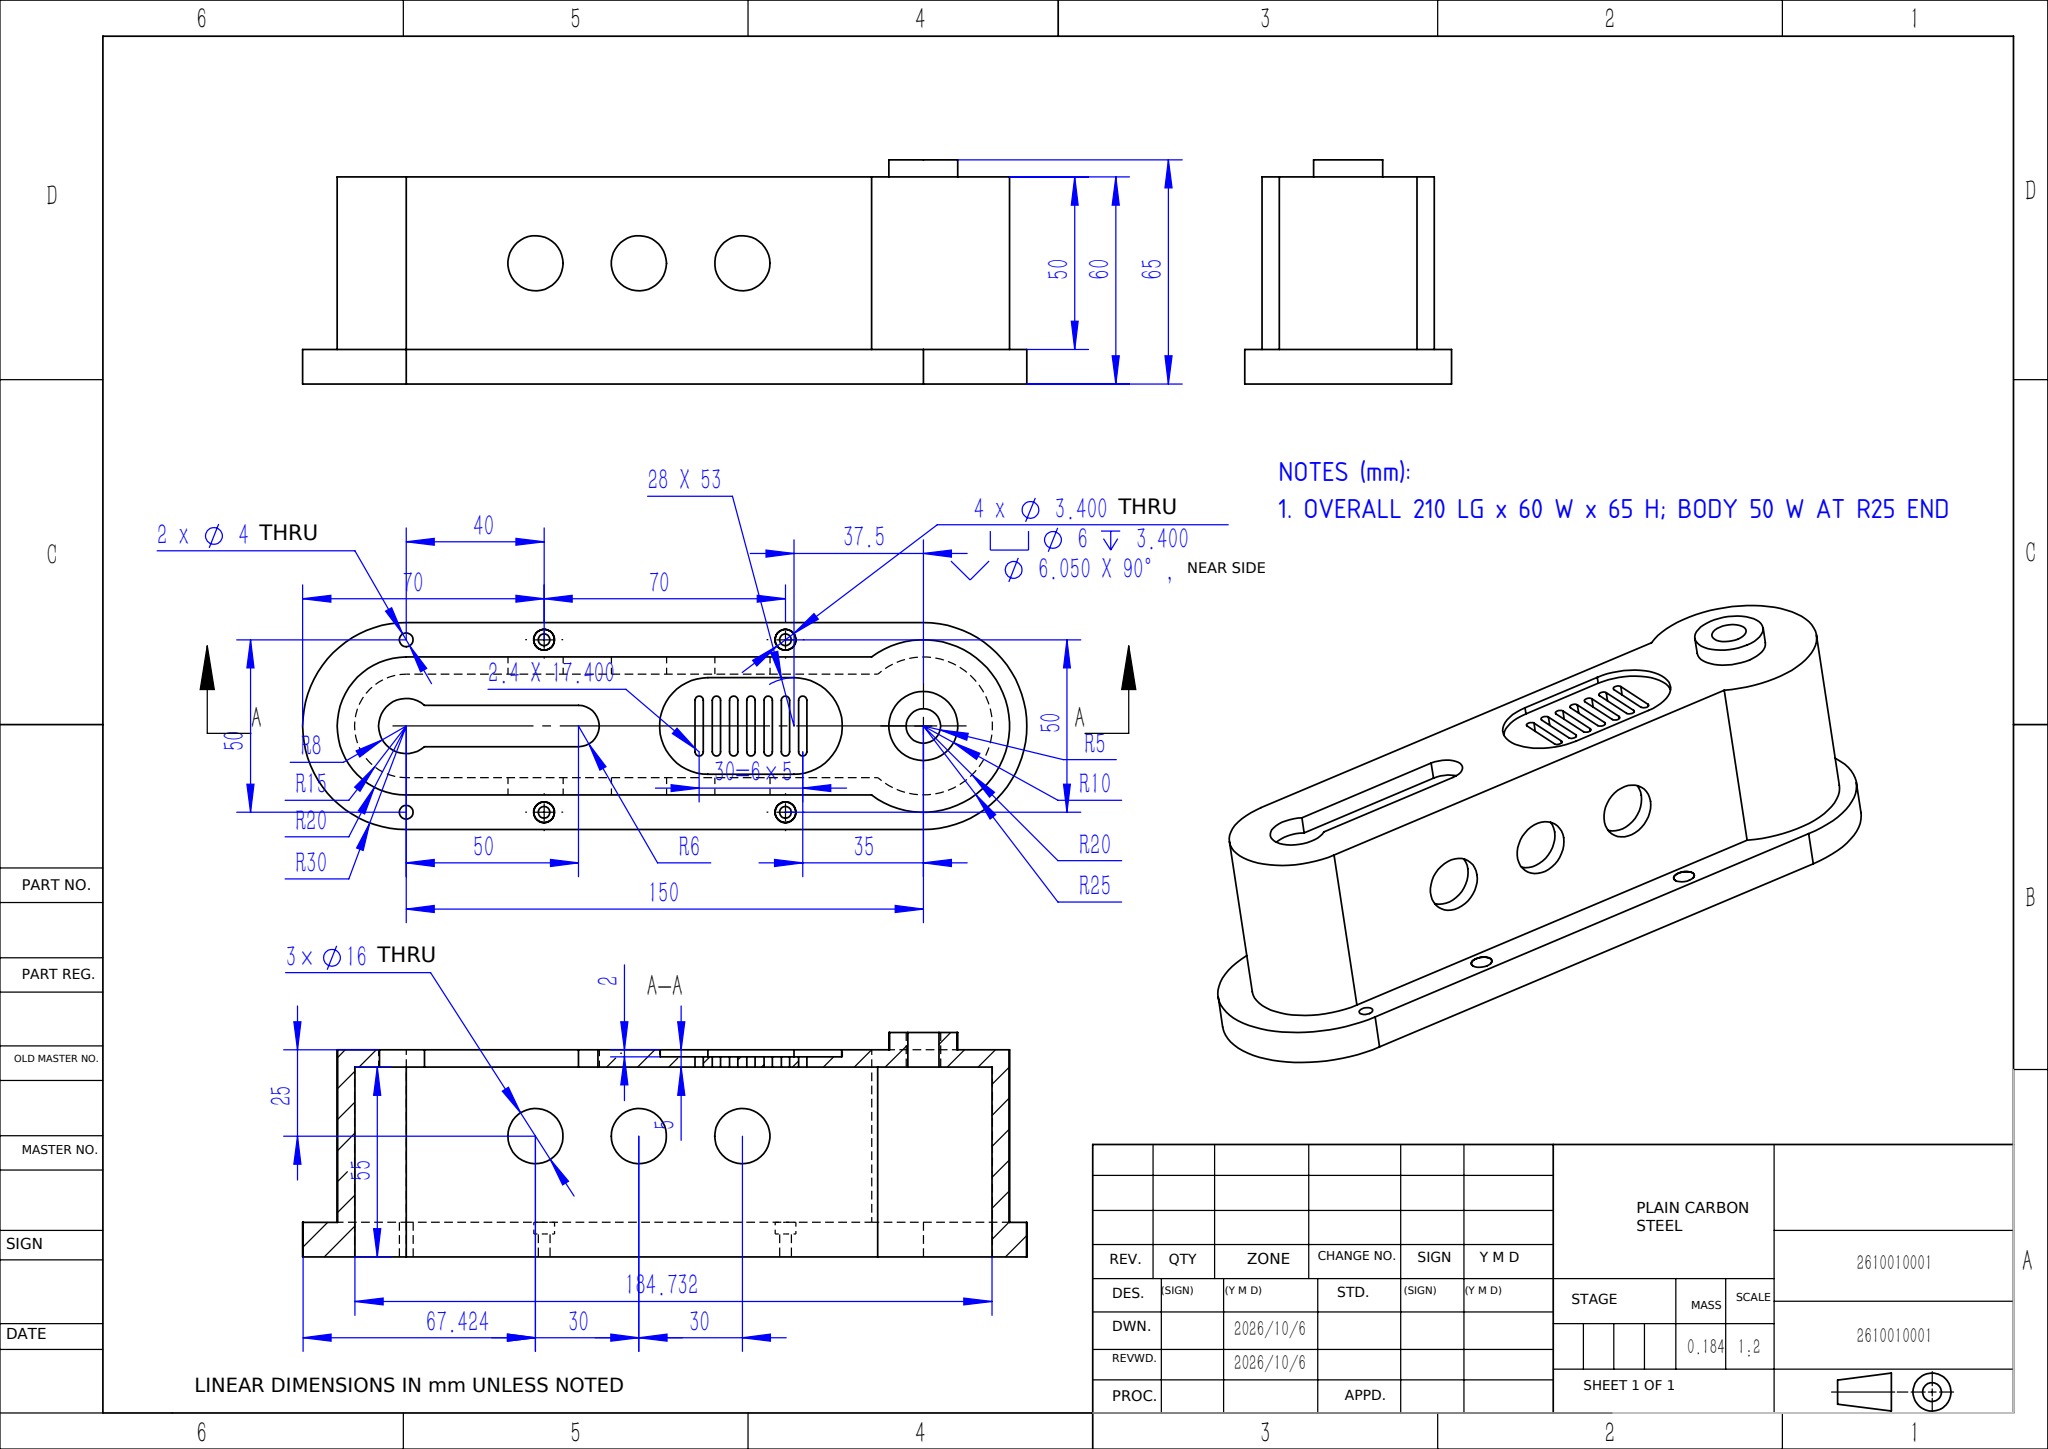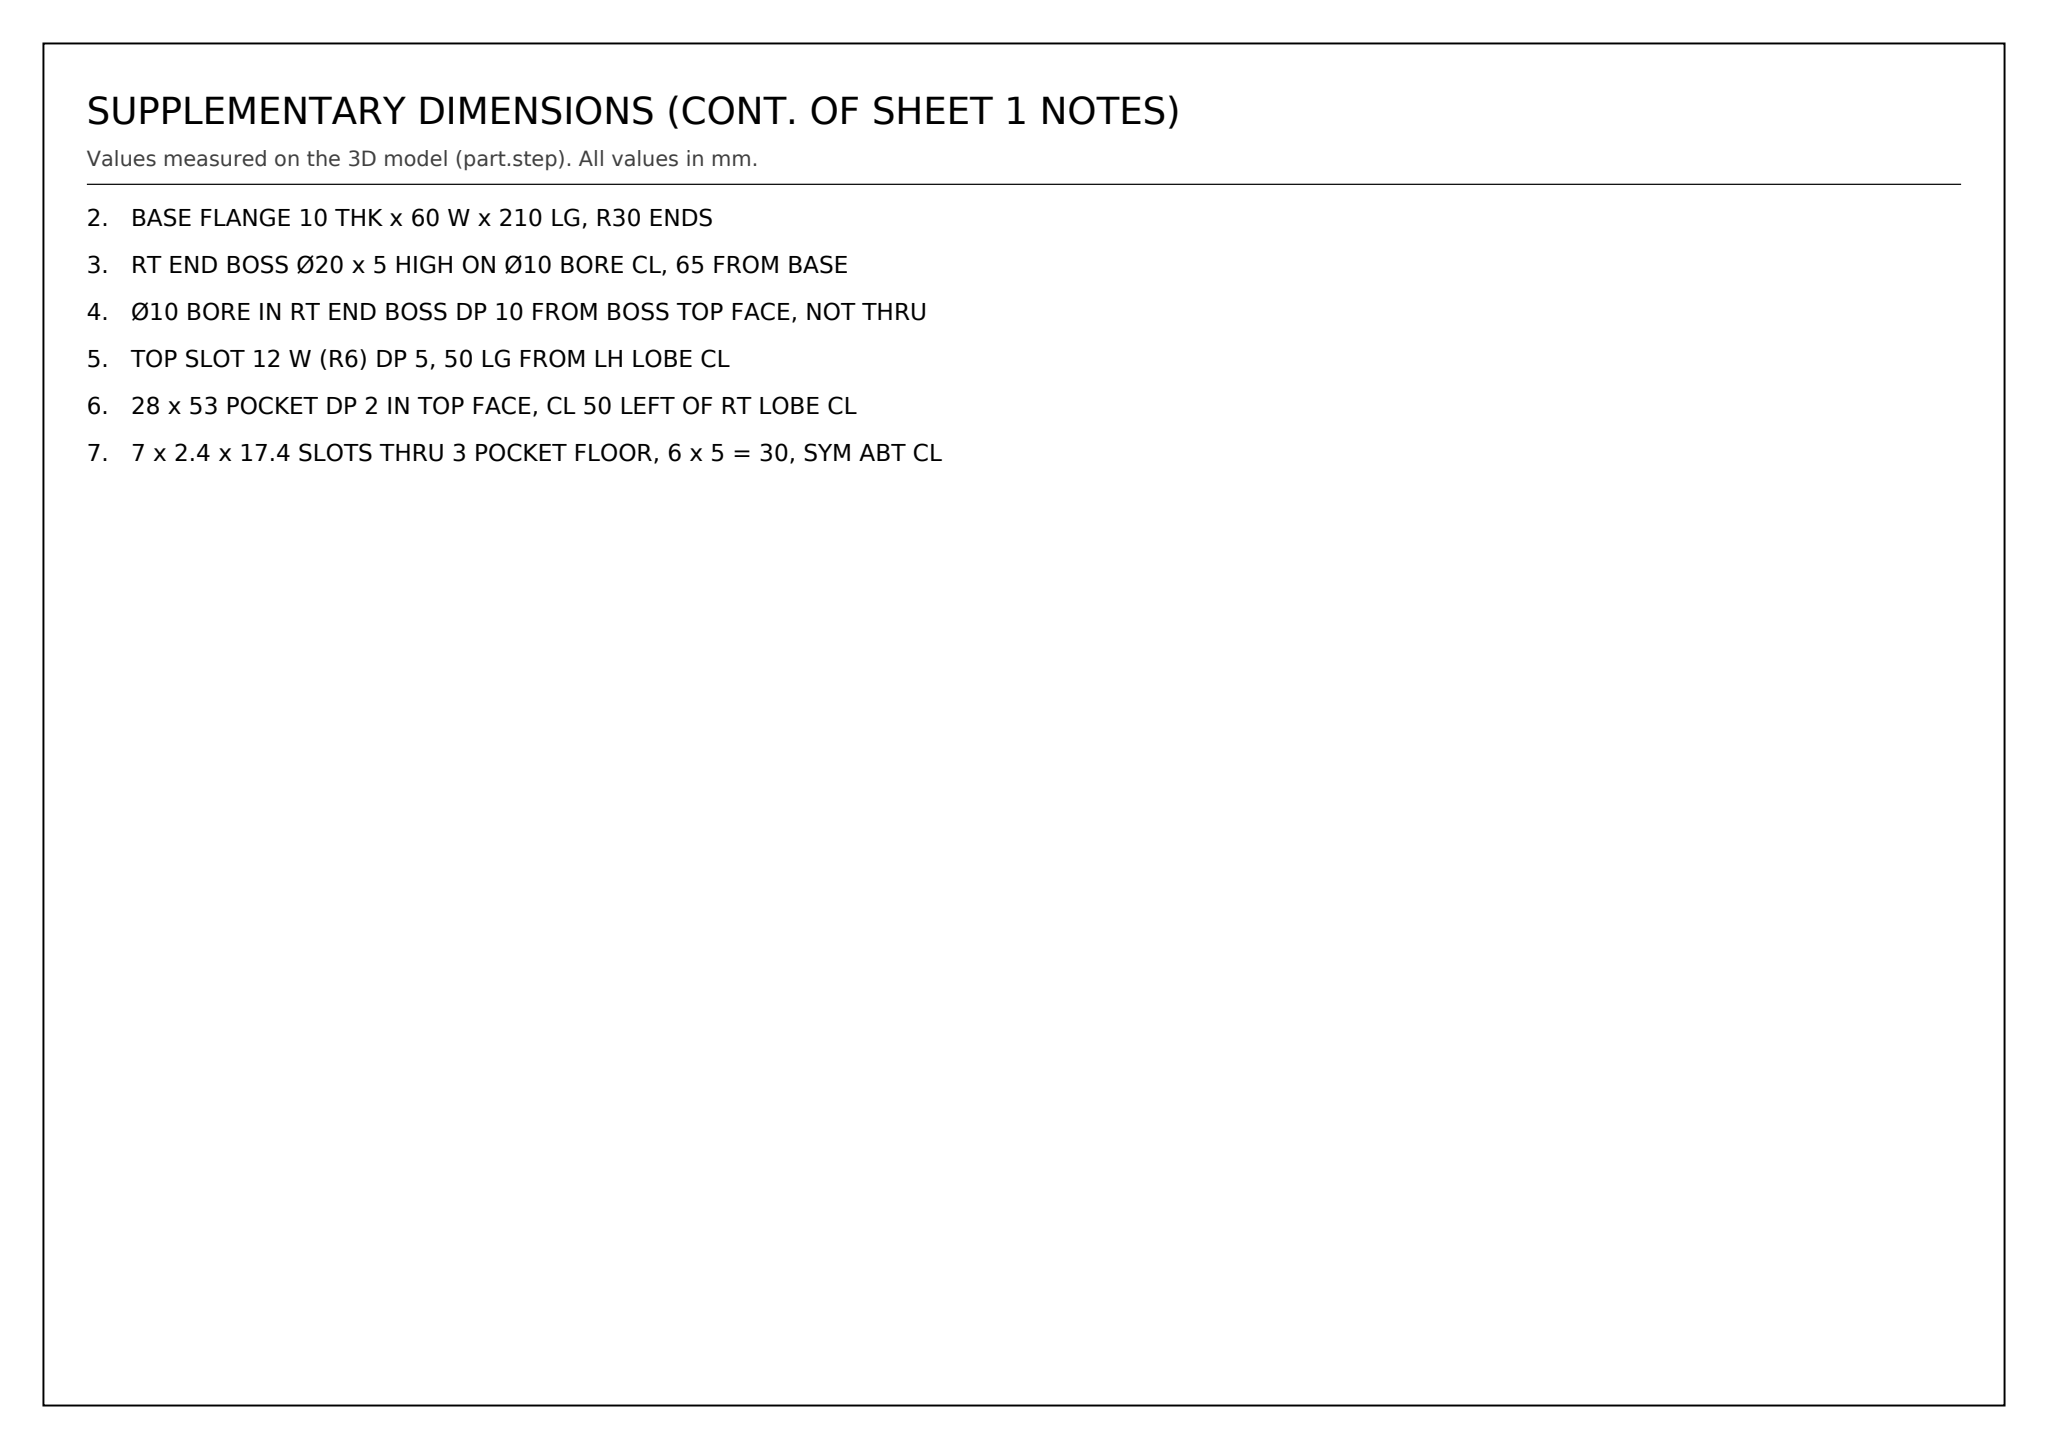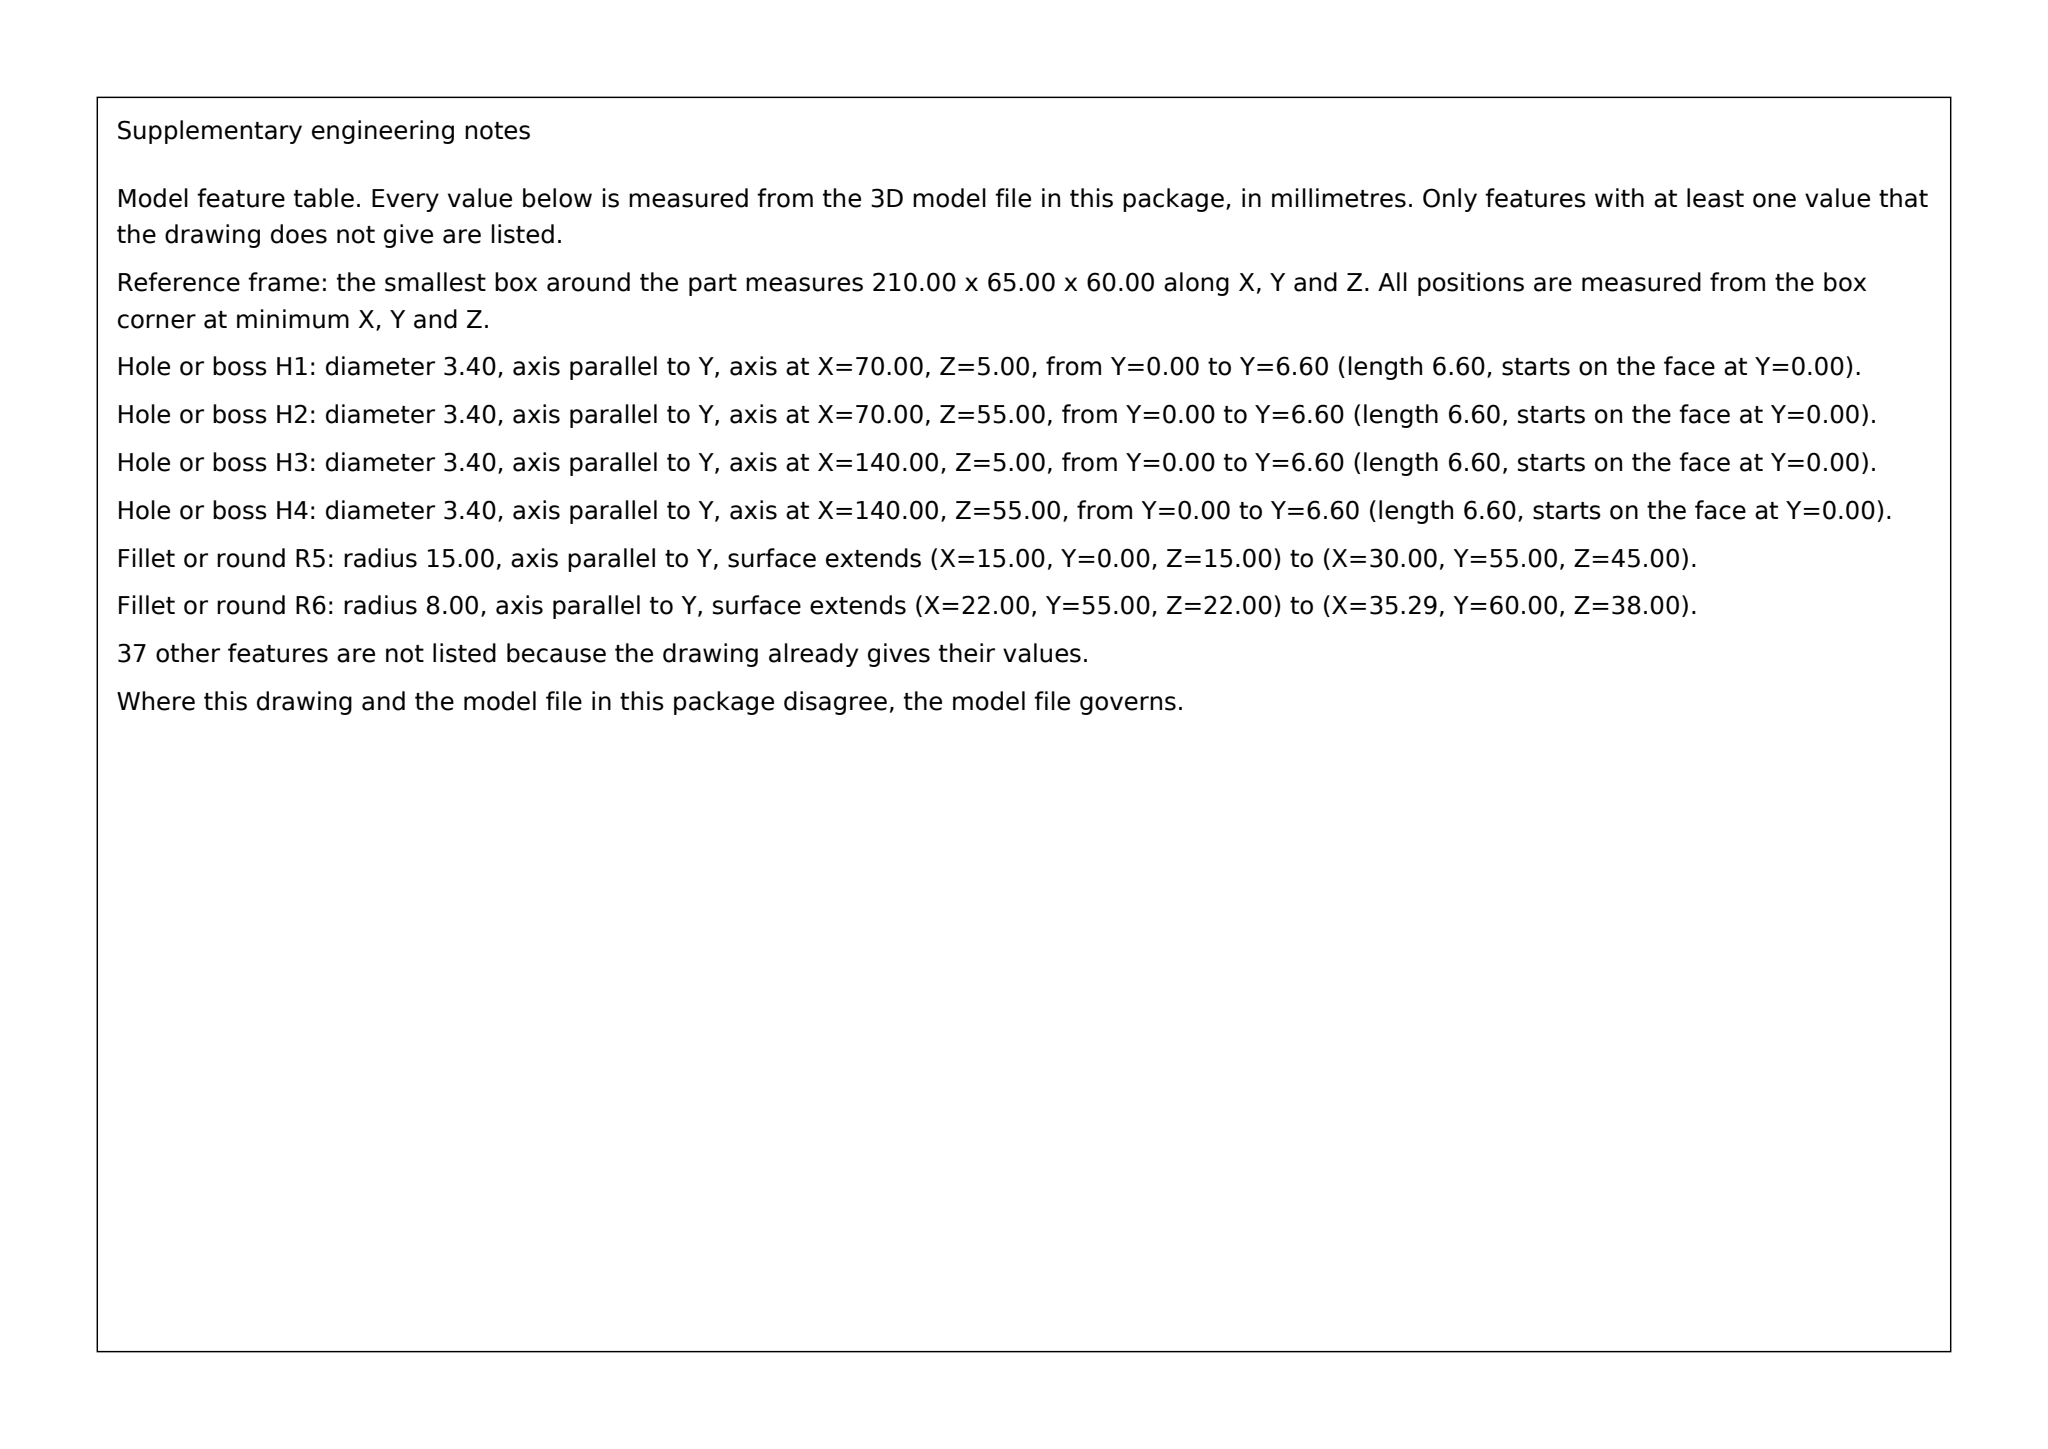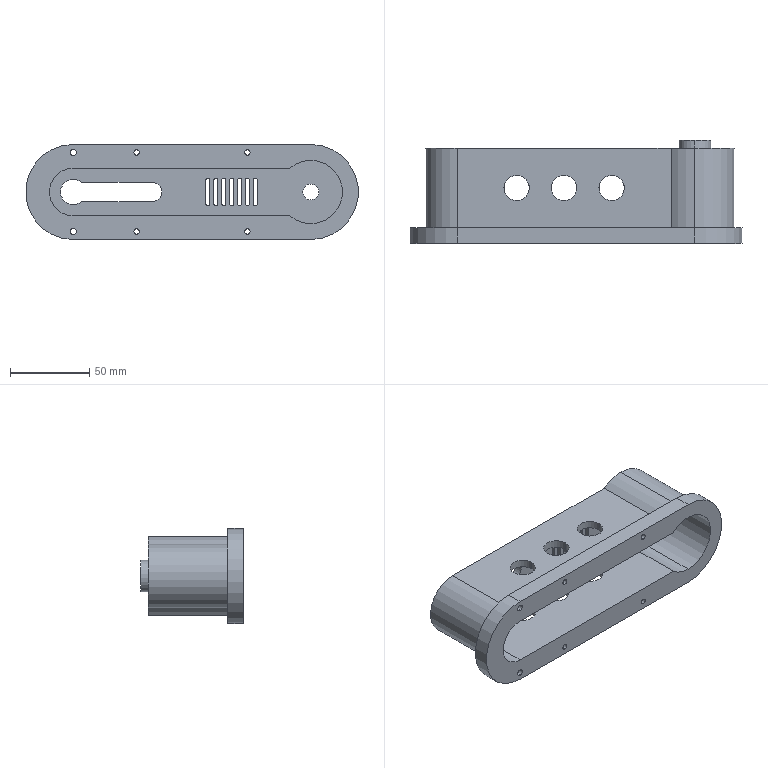Part | SolidWorks | mm | 1 solid | 115 faces | box 210 x 65 x 60 mm | volume 183942 mm3 | cylinder 73 | plane 34 | cone 8 | commonest cylinder face diameters 2.4 x21 16 x15 6 x8 3.4 x8 4 x4 40 x4 50 x3 10 x2
Drawing notes:
OVERALL 210 LG x 60 W x 65 H; BODY 50 W AT R25 END | from the solid: bbox 210 x 65 x 60; Ø60 and Ø50 y-cyls at z=30
BASE FLANGE 10 THK x 60 W x 210 LG, R30 ENDS | from the solid: Ø60 y-cyl len 10 at x=30 & x=180; y planes 0/10; bbox X=210
RT END BOSS Ø20 x 5 HIGH ON Ø10 BORE CL, 65 FROM BASE | from the solid: Ø20 y-cyl len 5 at x=180,z=30; y planes 60/65
Ø10 BORE IN RT END BOSS DP 10 FROM BOSS TOP FACE, NOT THRU | from the solid: cyl [10,"y",[180,null,30],len 10]; bore y=55..65
TOP SLOT 12 W (R6) DP 5, 50 LG FROM LH LOBE CL | from the solid: Ø12 y-cyl len 5 at x=80 and Ø16 y-cyl len 5 at x=30, z=30; y 55-60
28 x 53 POCKET DP 2 IN TOP FACE, CL 50 LEFT OF RT LOBE CL | from the solid: Ø28 y-cyls len 2 at x=117.5 & 142.5, z=30; y 58-60; CL x=130 vs 180
7 x 2.4 x 17.4 SLOTS THRU 3 POCKET FLOOR, 6 x 5 = 30, SYM ABT CL | from the solid: Ø2.4 y-cyls len 3 at x=115..145 step 5, z=22.5/37.5; y 55-58
build123d program:
from build123d import *

# Parameters (mm, degrees)
BOSS_EXTRUDE1_DEPTH                            = 10
BOSS_EXTRUDE2_DEPTH                            = 50
SKETCH4_R                                      = 10
BOSS_EXTRUDE3_DEPTH                            = 5
SKETCH5_R                                      = 5
CUT_EXTRUDE1_DEPTH                             = 128.083
CUT_EXTRUDE2_START                             = -5
CUT_EXTRUDE2_DEPTH                             = 120.599
M3_HEX_SOCKET_HEAD_CAP_SCREW_CBORE1_AT_2_COUNT = 2
M3_HEX_SOCKET_HEAD_CAP_SCREW_CBORE1_AT_2_PITCH = 70
M3_HEX_SOCKET_HEAD_CAP_SCREW_CBORE1_AT_3_COUNT = 2
M3_HEX_SOCKET_HEAD_CAP_SCREW_CBORE1_AT_3_PITCH = 50
M3_HEX_SOCKET_HEAD_CAP_SCREW_CBORE1_AT_4_COUNT = 2
M3_HEX_SOCKET_HEAD_CAP_SCREW_CBORE1_AT_4_PITCH = 86.023
CUT_EXTRUDE3_DEPTH                             = 125.599
CUT_EXTRUDE4_DEPTH                             = 2
CUT_EXTRUDE6_REACH                             = 125.649
F_4_0_4_DIAMETER_HOLE1_D                       = 4
SKETCH18_R                                     = 8
CUT_EXTRUDE7_DEPTH                             = 134.229


with BuildPart() as part:
    # Sketch1 → Boss-Extrude1 (new body)
    with BuildSketch(Plane(origin=(0, 0, 0), x_dir=(1, 0, 0), z_dir=(0, 1, 0))):
        with BuildLine():
            Line((-75, 30), (75, 30))
            ThreePointArc((75, 30), (105, 0), (75, -30))
            Line((75, -30), (-75, -30))
            ThreePointArc((-75, -30), (-105, 0), (-75, 30))
        make_face()
    extrude(amount=BOSS_EXTRUDE1_DEPTH)

    # Sketch2 → Boss-Extrude2 (add)
    with BuildSketch(Plane(origin=(0, 10, 0), x_dir=(1, 0, 0), z_dir=(0, 1, 0))):
        with BuildLine():
            Line((-75, -20), (60, -20))
            ThreePointArc((60, -20), (100, 0), (60, 20))
            Line((60, 20), (-75, 20))
            ThreePointArc((-75, 20), (-95, 0), (-75, -20))
        make_face()
    extrude(amount=BOSS_EXTRUDE2_DEPTH)

    # Sketch4 → Boss-Extrude3 (add)
    with BuildSketch(Plane(origin=(0, 60, 0), x_dir=(1, 0, 0), z_dir=(0, 1, 0))):
        with Locations(Location((75, 0, 0), (0, 0, 270))):
            Circle(SKETCH4_R)
    extrude(amount=BOSS_EXTRUDE3_DEPTH)

    # Sketch5 → Cut-Extrude1 (cut, through all)
    with BuildSketch(Plane(origin=(0, 65, 0), x_dir=(1, 0, 0), z_dir=(0, 1, 0))):
        with Locations(Location((75, 0, 0), (0, 0, 270))):
            Circle(SKETCH5_R)
    extrude(amount=-CUT_EXTRUDE1_DEPTH, mode=Mode.SUBTRACT)

    # Sketch6 → Cut-Extrude2 (cut, through all)
    with BuildSketch(Plane(origin=(0, 60, 0), x_dir=(1, 0, 0), z_dir=(0, 1, 0)).offset(CUT_EXTRUDE2_START)):
        with BuildLine():
            Line((61.771, 15), (-75, 15))
            ThreePointArc((-75, 15), (-90, 0), (-75, -15))
            Line((-75, -15), (61.771, -15))
            ThreePointArc((61.771, -15), (95, 0), (61.771, 15))
        make_face()
    extrude(amount=-CUT_EXTRUDE2_DEPTH, mode=Mode.SUBTRACT)

    # Sketch8 → M3 Hex Socket Head Cap Screw CBORE1 (revolve, cut)
    with BuildSketch(Plane(origin=(-35, 10, 25), x_dir=(0, 0, 1), z_dir=(1, 0, 0))):
        Polygon((0, 0), (0, 10), (1.7, 10), (1.7, 3.4), (3, 3.4), (3, 0.025), (3.025, 0), align=None)
    m3_hex_socket_head_cap_screw_cbore1 = revolve(axis=Axis((-35, 16.35, 25), (0, -1, 0)), mode=Mode.SUBTRACT)

    # M3 Hex Socket Head Cap Screw CBORE1 at 2: M3 Hex Socket Head Cap Screw CBORE1 ×2
    with Locations(*[(i * M3_HEX_SOCKET_HEAD_CAP_SCREW_CBORE1_AT_2_PITCH, 0, 0) for i in range(1, M3_HEX_SOCKET_HEAD_CAP_SCREW_CBORE1_AT_2_COUNT)]):
        add(m3_hex_socket_head_cap_screw_cbore1, mode=Mode.SUBTRACT)

    # M3 Hex Socket Head Cap Screw CBORE1 at 3: M3 Hex Socket Head Cap Screw CBORE1 ×2
    with Locations(*[(0, 0, -i * M3_HEX_SOCKET_HEAD_CAP_SCREW_CBORE1_AT_3_PITCH) for i in range(1, M3_HEX_SOCKET_HEAD_CAP_SCREW_CBORE1_AT_3_COUNT)]):
        add(m3_hex_socket_head_cap_screw_cbore1, mode=Mode.SUBTRACT)

    # M3 Hex Socket Head Cap Screw CBORE1 at 4: M3 Hex Socket Head Cap Screw CBORE1 ×2
    with Locations(*[Vector(0.8137, 0, -0.5812) * (i * M3_HEX_SOCKET_HEAD_CAP_SCREW_CBORE1_AT_4_PITCH) for i in range(1, M3_HEX_SOCKET_HEAD_CAP_SCREW_CBORE1_AT_4_COUNT)]):
        add(m3_hex_socket_head_cap_screw_cbore1, mode=Mode.SUBTRACT)

    # Sketch12 → Cut-Extrude3 (cut, through all)
    with BuildSketch(Plane(origin=(0, 60, 0), x_dir=(1, 0, 0), z_dir=(0, 1, 0))):
        with BuildLine():
            Line((-69.708, 6), (-25, 6))
            ThreePointArc((-25, 6), (-19, 0), (-25, -6))
            Line((-25, -6), (-69.708, -6))
            ThreePointArc((-69.708, -6), (-83, 0), (-69.708, 6))
        make_face()
    extrude(amount=-CUT_EXTRUDE3_DEPTH, mode=Mode.SUBTRACT)

    # Sketch13 → Cut-Extrude4 (cut)
    with BuildSketch(Plane(origin=(0, 60, 0), x_dir=(1, 0, 0), z_dir=(0, 1, 0))):
        with BuildLine():
            Line((12.5, 14), (37.5, 14))
            ThreePointArc((37.5, 14), (51.5, 0), (37.5, -14))
            Line((37.5, -14), (12.5, -14))
            ThreePointArc((12.5, -14), (-1.5, 0), (12.5, 14))
        make_face()
    extrude(amount=-CUT_EXTRUDE4_DEPTH, mode=Mode.SUBTRACT)

    # Sketch14 → Cut-Extrude6 (cut, up to next)
    with BuildSketch(Plane(origin=(0, 58, 0), x_dir=(1, 0, 0), z_dir=(0, 1, 0)), mode=Mode.PRIVATE) as cut_extrude6_sk1:
        with BuildLine():
            Line((41.2, 7.5), (41.2, -7.5))
            ThreePointArc((41.2, -7.5), (40, -8.7), (38.8, -7.5))
            Line((38.8, -7.5), (38.8, 7.5))
            ThreePointArc((38.8, 7.5), (40, 8.7), (41.2, 7.5))
        make_face()
    cut_extrude6_tool1 = extrude(cut_extrude6_sk1.sketch, amount=-CUT_EXTRUDE6_REACH, mode=Mode.PRIVATE) & part.part
    # Sketch14 → Cut-Extrude6 (cut, up to next)
    with BuildSketch(Plane(origin=(0, 58, 0), x_dir=(1, 0, 0), z_dir=(0, 1, 0)), mode=Mode.PRIVATE) as cut_extrude6_sk2:
        with BuildLine():
            Line((36.2, 7.5), (36.2, -7.5))
            ThreePointArc((36.2, -7.5), (35, -8.7), (33.8, -7.5))
            Line((33.8, -7.5), (33.8, 7.5))
            ThreePointArc((33.8, 7.5), (35, 8.7), (36.2, 7.5))
        make_face()
    cut_extrude6_tool2 = extrude(cut_extrude6_sk2.sketch, amount=-CUT_EXTRUDE6_REACH, mode=Mode.PRIVATE) & part.part
    # Sketch14 → Cut-Extrude6 (cut, up to next)
    with BuildSketch(Plane(origin=(0, 58, 0), x_dir=(1, 0, 0), z_dir=(0, 1, 0)), mode=Mode.PRIVATE) as cut_extrude6_sk3:
        with BuildLine():
            Line((31.2, 7.5), (31.2, -7.5))
            ThreePointArc((31.2, -7.5), (30, -8.7), (28.8, -7.5))
            Line((28.8, -7.5), (28.8, 7.5))
            ThreePointArc((28.8, 7.5), (30, 8.7), (31.2, 7.5))
        make_face()
    cut_extrude6_tool3 = extrude(cut_extrude6_sk3.sketch, amount=-CUT_EXTRUDE6_REACH, mode=Mode.PRIVATE) & part.part
    # Sketch14 → Cut-Extrude6 (cut, up to next)
    with BuildSketch(Plane(origin=(0, 58, 0), x_dir=(1, 0, 0), z_dir=(0, 1, 0)), mode=Mode.PRIVATE) as cut_extrude6_sk4:
        with BuildLine():
            Line((26.2, 7.5), (26.2, -7.5))
            ThreePointArc((26.2, -7.5), (25, -8.7), (23.8, -7.5))
            Line((23.8, -7.5), (23.8, 7.5))
            ThreePointArc((23.8, 7.5), (25, 8.7), (26.2, 7.5))
        make_face()
    cut_extrude6_tool4 = extrude(cut_extrude6_sk4.sketch, amount=-CUT_EXTRUDE6_REACH, mode=Mode.PRIVATE) & part.part
    # Sketch14 → Cut-Extrude6 (cut, up to next)
    with BuildSketch(Plane(origin=(0, 58, 0), x_dir=(1, 0, 0), z_dir=(0, 1, 0)), mode=Mode.PRIVATE) as cut_extrude6_sk5:
        with BuildLine():
            Line((21.2, 7.5), (21.2, -7.5))
            ThreePointArc((21.2, -7.5), (20, -8.7), (18.8, -7.5))
            Line((18.8, -7.5), (18.8, 7.5))
            ThreePointArc((18.8, 7.5), (20, 8.7), (21.2, 7.5))
        make_face()
    cut_extrude6_tool5 = extrude(cut_extrude6_sk5.sketch, amount=-CUT_EXTRUDE6_REACH, mode=Mode.PRIVATE) & part.part
    # Sketch14 → Cut-Extrude6 (cut, up to next)
    with BuildSketch(Plane(origin=(0, 58, 0), x_dir=(1, 0, 0), z_dir=(0, 1, 0)), mode=Mode.PRIVATE) as cut_extrude6_sk6:
        with BuildLine():
            Line((16.2, 7.5), (16.2, -7.5))
            ThreePointArc((16.2, -7.5), (15, -8.7), (13.8, -7.5))
            Line((13.8, -7.5), (13.8, 7.5))
            ThreePointArc((13.8, 7.5), (15, 8.7), (16.2, 7.5))
        make_face()
    cut_extrude6_tool6 = extrude(cut_extrude6_sk6.sketch, amount=-CUT_EXTRUDE6_REACH, mode=Mode.PRIVATE) & part.part
    # Sketch14 → Cut-Extrude6 (cut, up to next)
    with BuildSketch(Plane(origin=(0, 58, 0), x_dir=(1, 0, 0), z_dir=(0, 1, 0)), mode=Mode.PRIVATE) as cut_extrude6_sk7:
        with BuildLine():
            Line((11.2, 7.5), (11.2, -7.5))
            ThreePointArc((11.2, -7.5), (10, -8.7), (8.8, -7.5))
            Line((8.8, -7.5), (8.8, 7.5))
            ThreePointArc((8.8, 7.5), (10, 8.7), (11.2, 7.5))
        make_face()
    cut_extrude6_tool7 = extrude(cut_extrude6_sk7.sketch, amount=-CUT_EXTRUDE6_REACH, mode=Mode.PRIVATE) & part.part
    add(cut_extrude6_tool1.solids().sort_by_distance((40, 58, 0))[0], mode=Mode.SUBTRACT)
    add(cut_extrude6_tool2.solids().sort_by_distance((35, 58, 0))[0], mode=Mode.SUBTRACT)
    add(cut_extrude6_tool3.solids().sort_by_distance((30, 58, 0))[0], mode=Mode.SUBTRACT)
    add(cut_extrude6_tool4.solids().sort_by_distance((25, 58, 0))[0], mode=Mode.SUBTRACT)
    add(cut_extrude6_tool5.solids().sort_by_distance((20, 58, 0))[0], mode=Mode.SUBTRACT)
    add(cut_extrude6_tool6.solids().sort_by_distance((15, 58, 0))[0], mode=Mode.SUBTRACT)
    add(cut_extrude6_tool7.solids().sort_by_distance((10, 58, 0))[0], mode=Mode.SUBTRACT)

    # 4.0 _4_ Diameter Hole1 (through all)
    with Locations(Plane(origin=(0, 10, 0), x_dir=(1, 0, 0), z_dir=(0, 1, 0))):
        with Locations((-75, 25), (-75, -25)):
            Hole(F_4_0_4_DIAMETER_HOLE1_D / 2)

    # Sketch18 → Cut-Extrude7 (cut, through all)
    with BuildSketch(Plane.XY.offset(20)):
        with Locations((-37.5, 35)):
            Circle(SKETCH18_R)
        with Locations((-7.5, 35)):
            Circle(SKETCH18_R)
        with Locations((22.5, 35)):
            Circle(SKETCH18_R)
    extrude(amount=-CUT_EXTRUDE7_DEPTH, mode=Mode.SUBTRACT)


solid = part.part